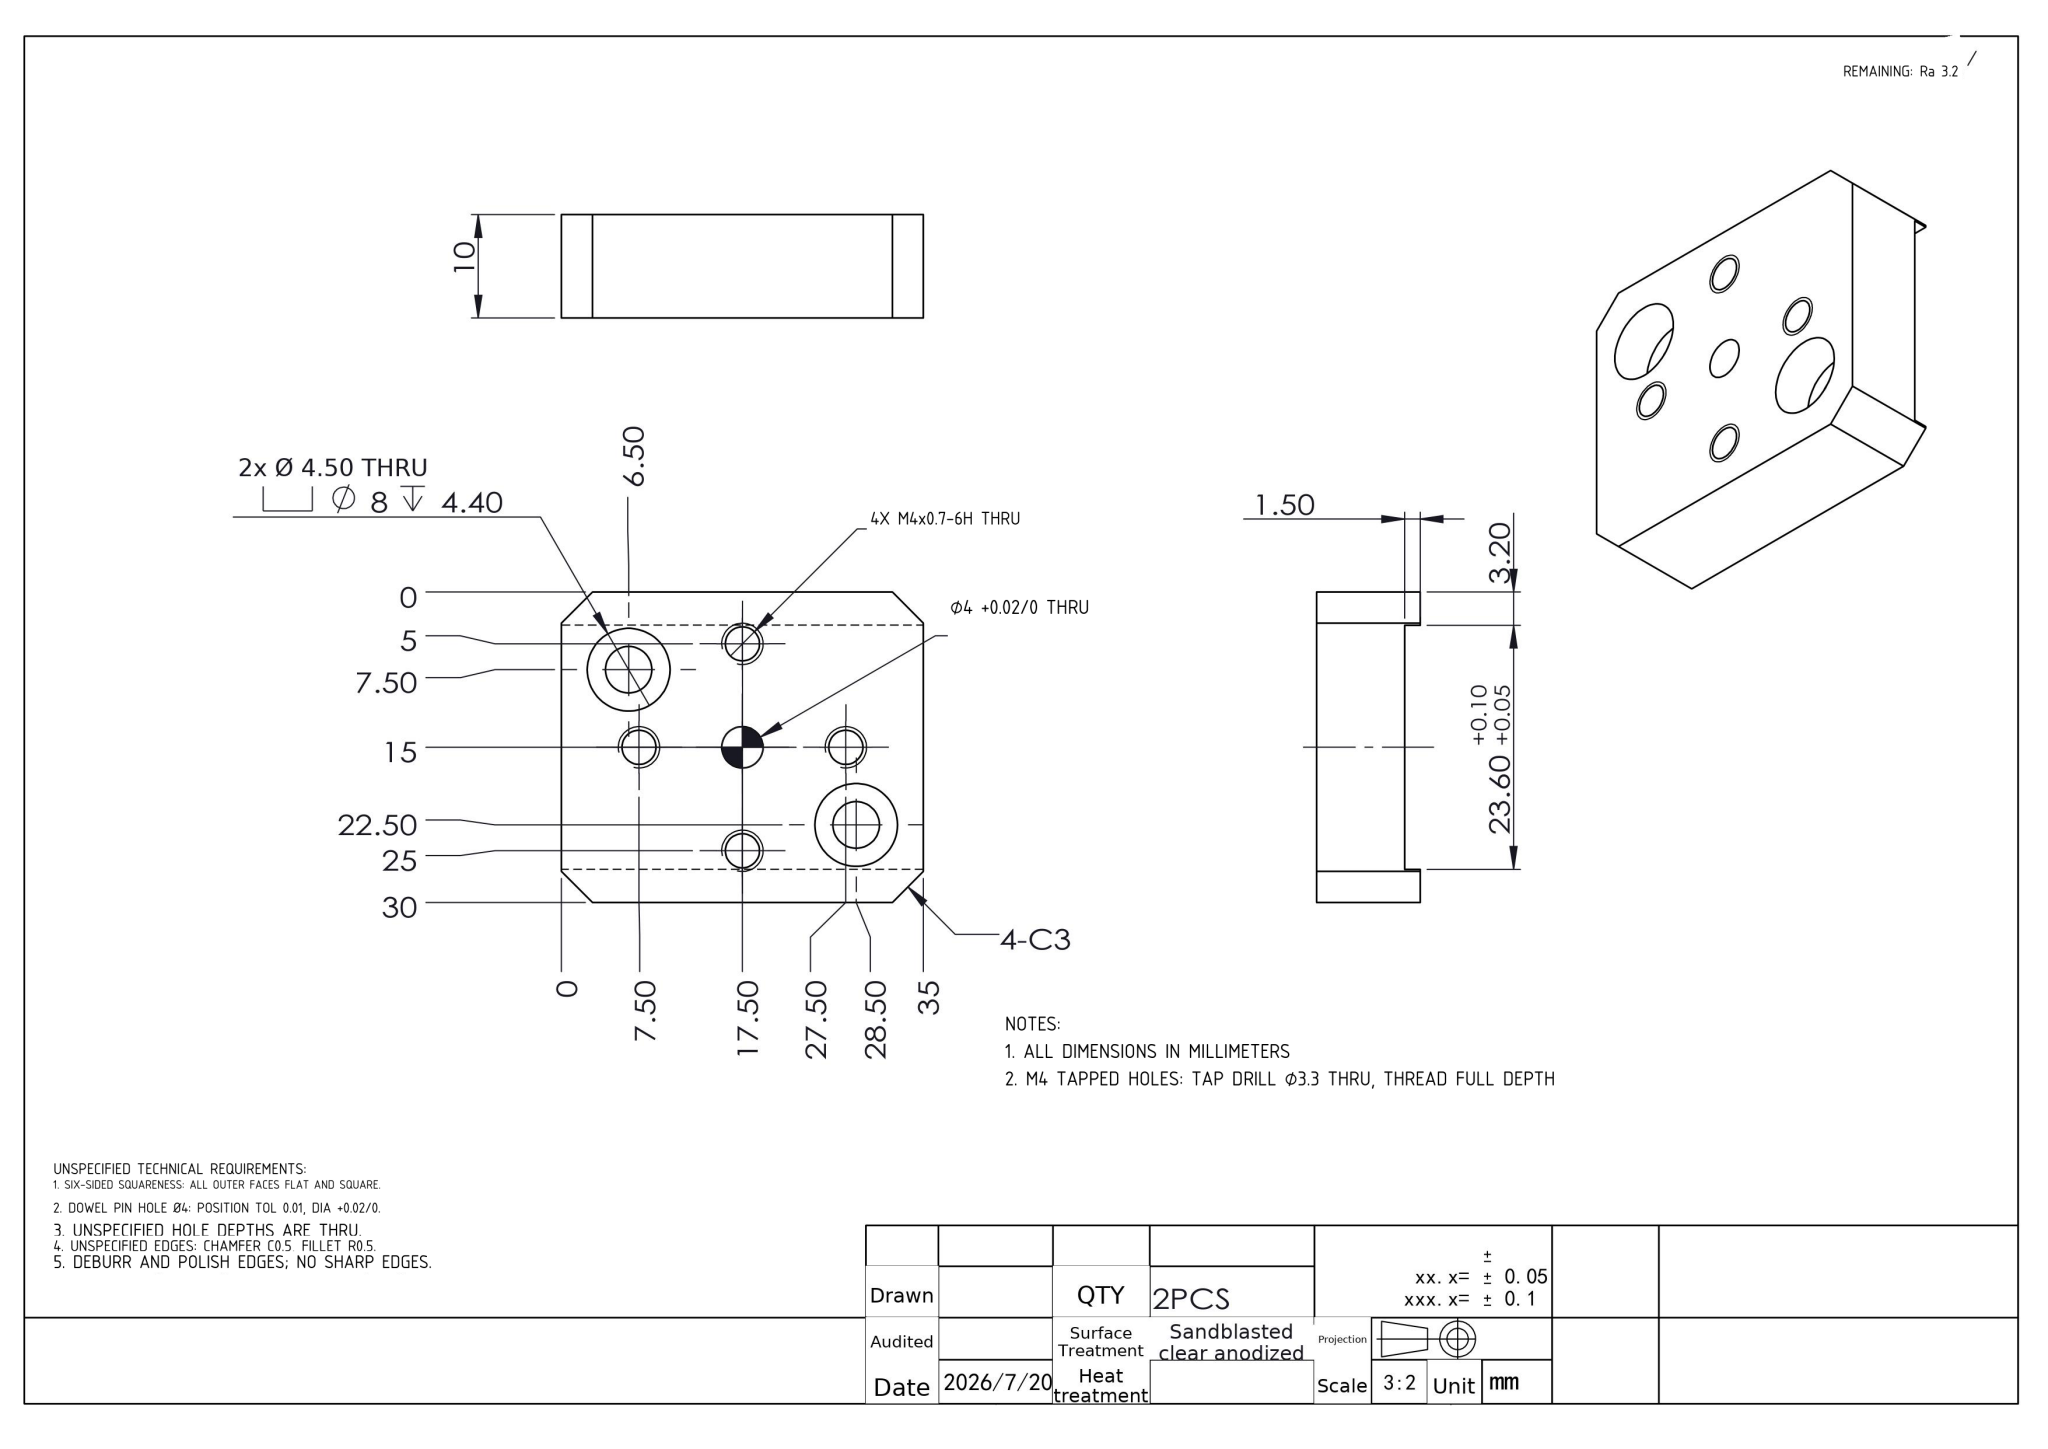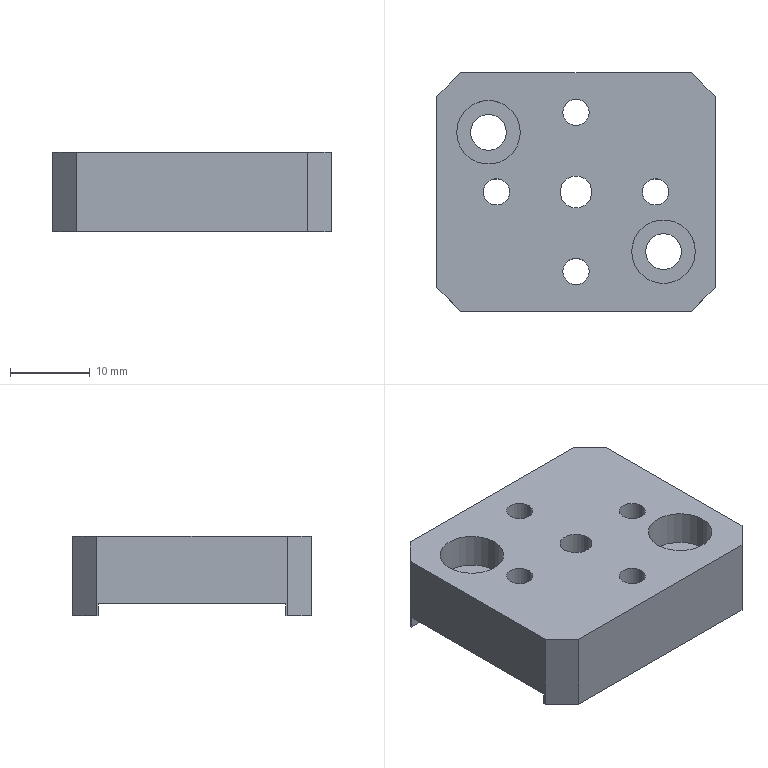Part | NX | mm | 1 solid | 34 faces | box 35 x 30 x 10 mm | volume 8111 mm3 | cylinder 18 | plane 16 | commonest cylinder face diameters 3.3 x8 8 x4 4.5 x4 4 x2